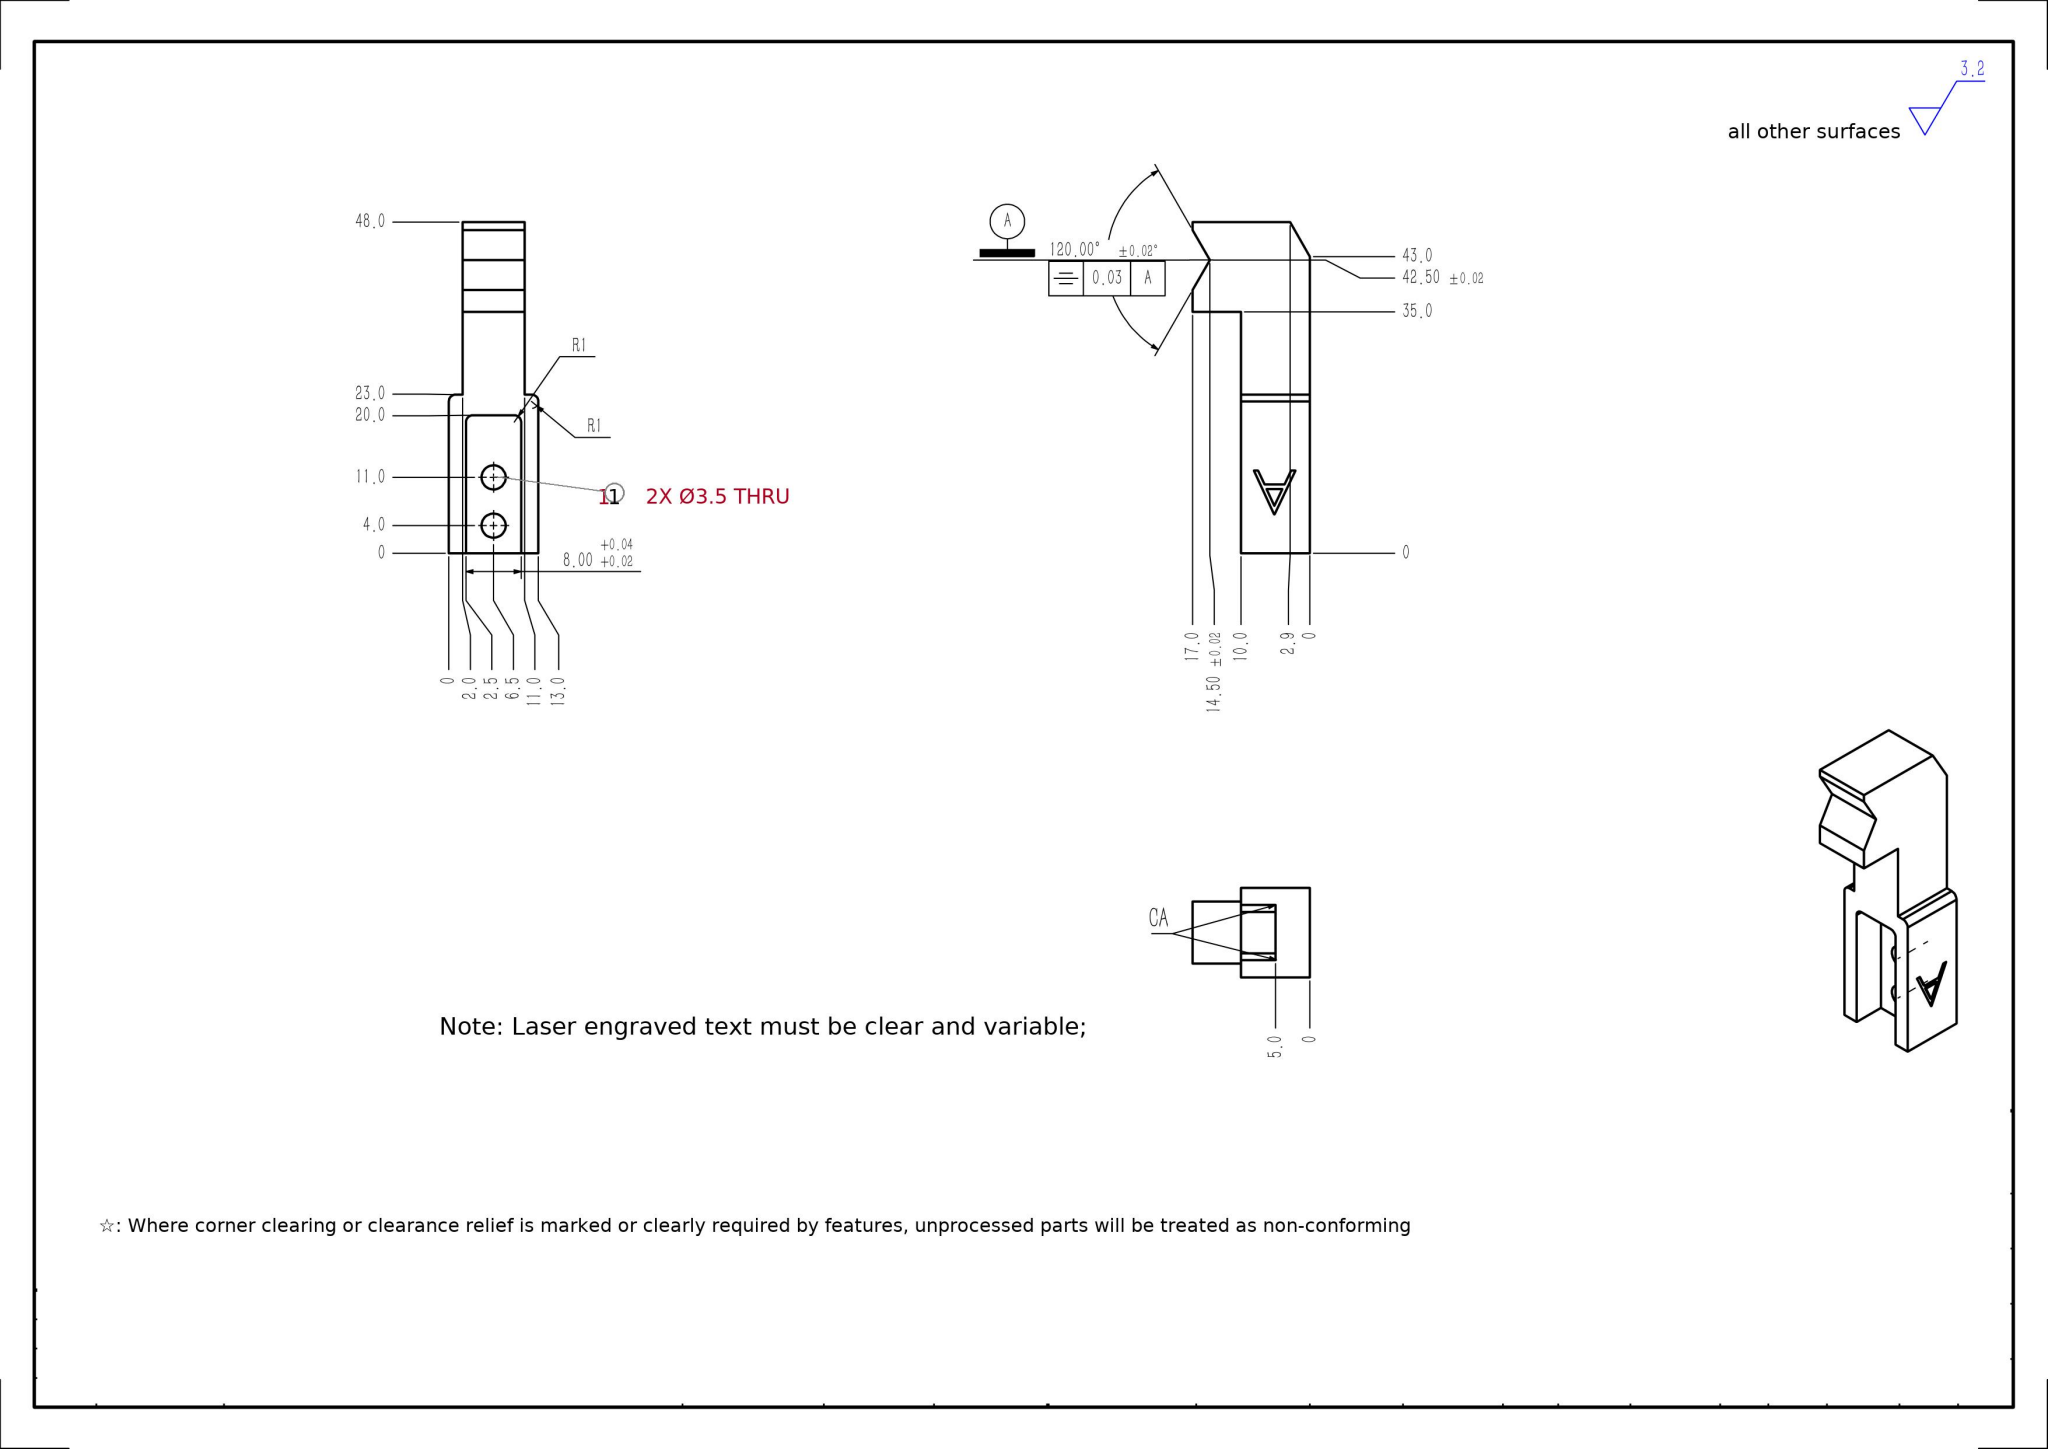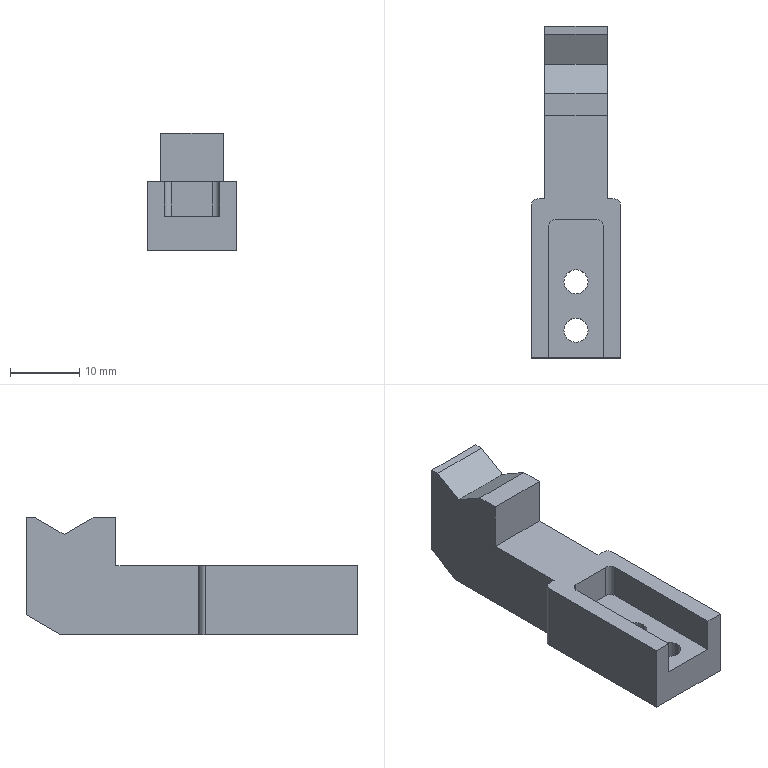Part | SolidWorks | mm | 1 solid | 41 faces | box 13 x 48 x 17 mm | volume 4996 mm3 | plane 33 | cylinder 8 | commonest cylinder face diameters 3.5 x4 2 x4
build123d program:
from build123d import *

# Parameters (mm, degrees)
SKETCH1_W                  = 20
SKETCH1_H                  = 48
BOSS_EXTRUDE1_DEPTH        = 5
SKETCH2_W                  = 8
SKETCH2_H                  = 40
CUT_EXTRUDE1_DEPTH         = 5
SKETCH3_W                  = 3.5
SKETCH3_H                  = 35
CUT_EXTRUDE2_DEPTH         = 28.857
SKETCH4_W                  = 20
SKETCH4_H                  = 13
BOSS_EXTRUDE2_DEPTH        = 8
F_3_5_3_5_DIAMETER_HOLE1_D = 3.5
SKETCH8_W                  = 20
SKETCH8_H                  = 13
CUT_EXTRUDE4_DEPTH         = 1
FILLET3_R                  = 1
SKETCH9_W                  = 5.5
SKETCH9_H                  = 25
CUT_EXTRUDE5_DEPTH         = 21
FILLET4_R                  = 1
CHAMFER3_SIZE              = 5
CHAMFER3_SIZE2             = 2.887
CUT_EXTRUDE6_DEPTH         = 30
CUT_EXTRUDE7_DEPTH         = 0.2


with BuildPart() as part:
    # Sketch1 → Boss-Extrude1 (new, symmetric)
    with BuildSketch(Plane.XY):
        Rectangle(SKETCH1_W, SKETCH1_H)
    extrude(amount=BOSS_EXTRUDE1_DEPTH, both=True)

    # Sketch2 → Cut-Extrude1 (cut)
    with BuildSketch(Plane.XY.offset(5)):
        with Locations((0, -24)):
            Rectangle(SKETCH2_W, SKETCH2_H)
    extrude(amount=-CUT_EXTRUDE1_DEPTH, mode=Mode.SUBTRACT)

    # Sketch3 → Cut-Extrude2 (cut, through all)
    with BuildSketch(Plane.XY.offset(5)):
        with Locations((-8.25, -6.5)):
            Rectangle(SKETCH3_W, SKETCH3_H)
        with Locations((8.25, -6.5)):
            Rectangle(SKETCH3_W, SKETCH3_H)
    extrude(amount=-CUT_EXTRUDE2_DEPTH, mode=Mode.SUBTRACT)

    # Sketch4 → Boss-Extrude2 (add)
    with BuildSketch(Plane.XY.offset(5)):
        with Locations((0, 17.5)):
            Rectangle(SKETCH4_W, SKETCH4_H)
    extrude(amount=BOSS_EXTRUDE2_DEPTH)

    # 3.5 _3.5_ Diameter Hole1 (through all)
    with Locations(Plane(origin=(0, 0, -5), x_dir=(-1, 0, 0), z_dir=(0, 0, -1))):
        with Locations((0, -20), (0, -13)):
            Hole(F_3_5_3_5_DIAMETER_HOLE1_D / 2)

    # Sketch8 → Cut-Extrude4 (cut)
    with BuildSketch(Plane.XY.offset(13)):
        with Locations((0, 17.5)):
            Rectangle(SKETCH8_W, SKETCH8_H)
    extrude(amount=-CUT_EXTRUDE4_DEPTH, mode=Mode.SUBTRACT)

    # Fillet3
    fillet3_edges = [part.edges().sort_by_distance(p)[0] for p in [
        (4, -4, 2.5),
        (-4, -4, 2.5),
    ]]
    fillet(fillet3_edges, radius=FILLET3_R)

    # Sketch9 → Cut-Extrude5 (cut)
    with BuildSketch(Plane(origin=(0, 0, -5), x_dir=(-1, 0, 0), z_dir=(0, 0, -1))):
        with Locations((-7.25, 11.5)):
            Rectangle(SKETCH9_W, SKETCH9_H)
    cut_extrude5 = extrude(amount=-CUT_EXTRUDE5_DEPTH, mode=Mode.SUBTRACT)

    # Mirror1: Cut-Extrude5 across plane
    add(cut_extrude5.mirror(Plane(origin=(0, 0, 0), x_dir=(0, 0, 1), z_dir=(1, 0, 0))), mode=Mode.SUBTRACT)

    # Fillet4
    fillet4_edges = [part.edges().sort_by_distance(p)[0] for p in [
        (6.5, -1, 0),
        (-6.5, -1, 0),
    ]]
    fillet(fillet4_edges, radius=FILLET4_R)

    # Chamfer3
    chamfer3_edges = [part.edges().sort_by_distance(p)[0] for p in [
        (0, 24, -5),
    ]]
    chamfer3_side = [part.faces().sort_by_distance(p)[0] for p in [
        (0, -1.65, -5),
    ]]
    chamfer(chamfer3_edges, length=CHAMFER3_SIZE, length2=CHAMFER3_SIZE2, reference=chamfer3_side[0])

    # Sketch10 → Cut-Extrude6 (cut, through all)
    with BuildSketch(Plane.ZY.offset(4.5)):
        Polygon((12, 14.17), (9.5, 18.5), (12, 22.83), align=None)
    extrude(amount=-CUT_EXTRUDE6_DEPTH, mode=Mode.SUBTRACT)

    # Sketch11 → Cut-Extrude7 (cut)
    with BuildSketch(Plane(origin=(6.5, 0, 0), x_dir=(0, 0, -1), z_dir=(1, 0, 0))):
        Polygon((-0.205, -18.35), (-3.136, -12), (-2.516, -12), (-1.577, -14.035), (1.301, -14.035), (2.267, -12), (2.889, -12), (-0.1236, -18.35), align=None)
        Polygon((-0.1579, -17.112), (0.992, -14.687), (-1.277, -14.687), align=None, mode=Mode.SUBTRACT)
    extrude(amount=-CUT_EXTRUDE7_DEPTH, mode=Mode.SUBTRACT)


solid = part.part